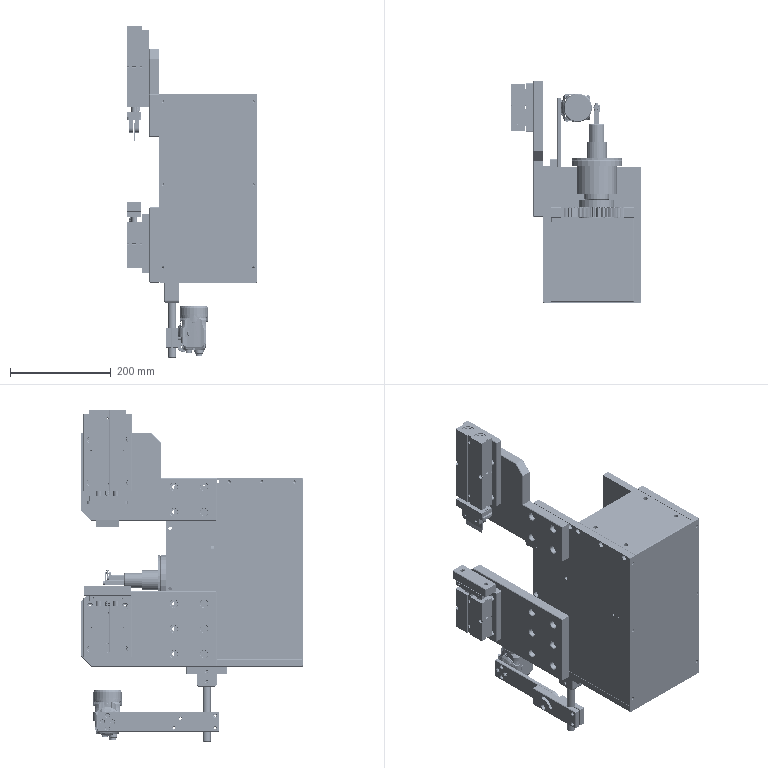Assembly | SolidWorks | mm | 54 component files | 54 solids | 5160 faces | box 260.2 x 442 x 660.5 mm | volume 8940176 mm3 | cylinder 1970 | plane 1868 | cone 912 | spline 408 | torus 2 | commonest cylinder face diameters 42 x148 8 x102 4 x85 0.4 x82 5 x74 11 x74 97.498 x70 111 x70
Bill of materials:
3M 35T | 1 | 1060 Alloy | Straight-tooth spur-gear-like disc with a cylindrical hub on one face and a keyed central bore.
BasePlate2 | 1 | 1060 Alloy | Thin rectangular, near-square plate with four through holes near the corners of the face and three holes in one edge face.
3M 35TS35B70H35L40 | 1 |  | Straight-tooth gear with a hub on one side, a large keyed bore and a ring of small holes in the web.
40ShaftRetainingRing | 1 |  | Thin flat split ring with two lugs at the gap, each with a small hole. The shape resembles an external retaining ring.
6008 GB 276-94 | 2 |  | Annular rolling-element-bearing-like assembly: an outer ring and an inner ring with a single row of balls between them.
68HoleRetainingRing | 2 |  | Thin flat open ring with two rounded lugs at the gap, each with a small hole. The shape resembles an internal retaining ring.
AirGripperFixingPlate1 | 1 | Plain Carbon Steel | Flat plate made of a circular disc joined to a rectangular tab, with a central rectangular cutout and several round holes.
AirGripperFixingPlate2 | 1 | 1060 Alloy | Rectangular block or thick plate with two round through holes.
BearingCoverPlate | 1 | Plain Carbon Steel | Thin flat annular disc with a large central hole and four small holes near the outer edge.
BearingHolder | 1 | Plain Carbon Steel | Flanged cylindrical sleeve: a hollow tube with a wider flange at one end that has a ring of holes.
Buckle | 1 |  | Push-in clip-like molded part: a wide winged head, a stem, a round disc flange, and a lower body with angled flexible-looking arms and a tip.
BuckleRotaryAxis | 1 | Plain Carbon Steel | Stepped cylindrical shaft with a raised collar, shallow ring grooves, and a rectangular socket in one end face surrounded by four small holes.
CylinderJaw1 | 1 | Plain Carbon Steel | Long straight square-section bar with an enlarged rectangular end block at one end, carrying four holes in a 2x2 pattern.
CylinderJaw2 | 1 | Plain Carbon Steel | Long straight rectangular-section bar with a rectangular end block at one end, carrying four holes in a 2x2 pattern; the block extends further below the bar than in the similar part.
FixedSleeve | 1 | Plain Carbon Steel | Short thin-walled cylindrical ring or sleeve with an open through-bore and small chamfers on the outer edges.
JawBuckleJaw | 1 | Plain Carbon Steel | Upright flat plate with a rounded top, an elongated slot near the top, a large round hole in the middle and a smaller round hole lower down; two parallel side flanges at the lower end give that section a U-channel shape.
JawBuckleJaw2 | 1 | Plain Carbon Steel | Shorter version of the flanged plate: rounded-top plate with an elongated slot above and one round hole below, and two parallel side flanges on the wider lower section forming a U-channel.
M4X16 | 3 |  | Fastener-like part: cylindrical head with a hexagonal socket recess, a short externally grooved (thread-like) section next to the head, then a longer smooth cylindrical shank of smaller diameter.
1_1_9 | 1 |  | Rectangular prismatic block with long grooves along its length, a central raised and stepped section, and several holes; the end face has two counterbored circular features.
2_13 | 1 |  | Square block plate with a large central through-hole and four corner holes, joined by a stepped offset web to a thin arm that extends sideways and ends in a small hooked lip.
3_10 | 1 |  | Square block plate with a large central hole and four corner holes, with a stepped side web and a thin arm extending the other way, ending in a small hooked lip.
SensorPlate3 | 1 | Plain Carbon Steel | L-shaped bent thin-sheet bracket with rounded outer corners and an elongated obround slot in one leg.
CameraFixingPlate | 1 | 1060 Alloy | Flat elongated plate with one fully rounded end and one square end, two holes near the rounded end and four holes in a diamond pattern near the square end.
GuideAxis16 | 1 | Plain Carbon Steel | Plain solid cylindrical rod or pin with small chamfers at both ends.
GuideAxisFixingPlate | 1 | 1060 Alloy | Stepped rectangular block with a split-clamp bore at one end and an arc slot through the thinner stepped section
GuideAxisHolder | 1 | 1060 Alloy | T-section block with a flange that has a large central bore and two flanking holes, and a downward web with two cross holes
IV-150_500_2000 | 1 |  | Complex housing with a rounded square body, a stepped circular top boss and cylindrical outlets at the bottom
OP-87436_87437 | 1 |  | Circular cap with a chamfered top, a circumferential groove and short legs or lobes below, one of which has a hole
OP-87460 | 1 |  | Curved, saddle-like bracket with a hole pattern on a central tab and a small angled flange with a hole
OP-87461 | 1 |  | Circular cap with a chamfered top, a circumferential groove, and downward legs, including a central lobe with a hole
CoverPlate4 | 1 | Plain Carbon Steel | Thin flat rectangular plate with six small holes along its two long edges
CutterBlade | 1 | Plain Carbon Steel | Flat rectangular blade-like plate with a bevel along one edge and two mounting holes
CutterFixingBlock | 1 | 1060 Alloy | Mounting bracket with a rounded-rectangle base plate and two parallel lugs with aligned cross holes
CutterFixingPlateA | 1 | 1060 Alloy | Flat rectangular plate with two chamfered corners, six larger holes and four smaller holes
CutterFixingPlateB | 1 | 1060 Alloy | L-outline flat plate with chamfered corners, four larger holes on the narrow leg and four smaller holes on the wide section
CutterNylonPad | 1 | 1060 Alloy | Rectangular block with chamfered edges and two counterbored or countersunk through-holes
Gasket5 | 1 | 1060 Alloy | Thick rectangular plate with a symmetric pattern of through holes: four larger holes and four smaller holes.
MHMJ082G1U_203 | 1 |  | Boxy body with a square flange that has four corner holes, a cylindrical shaft sticking out of one end, side-mounted connector-like housings with short bent cable stubs, and small screw heads on the end faces. Its overall form resembles a rotary motor.
SensorFixingBlock | 1 | Plain Carbon Steel | Thin L-shaped bent bracket. One leg has two round holes and the other leg has one large elongated (obround) slot.
ServoMotorFixingPlate | 1 | 1060 Alloy | Rectangular plate with a large central circular opening, four small holes around it, and four elongated slots near the short ends.
ServoMotorSideFixingPlate | 2 | 1060 Alloy | Square-section rectangular bar with two through holes on each of two adjacent faces, set at different heights.
ShimPlate4 | 1 | 1060 Alloy | Thick rectangular plate with four larger corner holes and four columns of five small holes each.
SideFixingPlate2 | 1 | 1060 Alloy | Thin flat plate with a stepped top edge (one corner area raised), two larger round holes, small holes next to them, and small holes along the top edge and side edge.
SideFixingPlate3 | 1 | 1060 Alloy | Tall rectangular block with two counterbored bores on the top end face, lengthwise grooves down the faces, T-shaped side slots, several through holes, and a small hex-shaped fitting sticking out of the bottom.
1_1_13 | 1 |  | Two parallel cylindrical rods standing on a rectangular base plate. Each rod ends in a larger-diameter cylindrical head.
2_17 | 1 |  | Shorter rectangular block with two large counterbored bores on top, a hex fitting and a small port next to them, lengthwise grooves, T-shaped side slots, and four through holes on the large face.
1_1_11 | 1 |  | Thin flat rectangular plate with many small holes in an irregular layout, grouped mostly toward one side and the top edge.
2_15 | 1 |  | Rectangular end plate holding two parallel cylindrical rods. Each rod ends in a larger cylindrical head, and the plate has two counterbored circular features and two small end holes.
TopCoverPlate | 1 | 1060 Alloy | Flat rectangular plate of uniform thickness with ten through holes: six slightly larger holes around the edge (one at each corner and one at the middle of each long edge) and four smaller plain holes set inward in an off-center rectangular pattern.
Mates:
1. coincident | BasePlate2-1 face at (-129.666, 120.264, 197.5) dir (-1, 0, 0) | SideFixingPlate3-1 face at (-129.666, 95.264, 197.5) dir (1, 0, 0)
2. concentric | BasePlate2-1 face at (-129.666, -24.736, 190) dir (-1, 0, 0) r 2.5 | SideFixingPlate3-1 face at (-144.666, -24.736, 190) dir (-1, 0, 0) r 3.3
3. concentric | BasePlate2-1 face at (-129.666, 105.264, 190) dir (-1, 0, 0) r 2.5 | SideFixingPlate3-1 face at (-144.666, 105.264, 190) dir (-1, 0, 0) r 5.5
4. coincident | BasePlate2-1 face at (35.334, 120.264, 197.5) dir (1, 0, 0) | SideFixingPlate2-1 face at (35.334, 87.764, 197.5) dir (-1, 0, 0)
5. concentric | BasePlate2-1 face at (35.334, -24.736, 190) dir (1, 0, 0) r 2.5 | SideFixingPlate2-1 face at (50.334, -24.736, 190) dir (1, 0, 0) r 5.5
6. concentric | BasePlate2-1 face at (35.334, 105.264, 190) dir (1, 0, 0) r 2.5 | SideFixingPlate2-1 face at (50.334, 105.264, 190) dir (1, 0, 0) r 5.5
7. coincident | SideFixingPlate2-1 face at (35.334, 87.764, 197.5) dir (-1, 0, 0) | ServoMotorSideFixingPlate-1 face at (35.334, 138.264, 99) dir (1, 0, 0)
8. concentric | SideFixingPlate2-1 face at (50.334, 138.264, 59) dir (1, 0, 0) r 3.4 | ServoMotorSideFixingPlate-1 face at (15.334, 138.264, 59) dir (-1, 0, 0) r 7.5
9. parallel | SideFixingPlate2-1 face at (50.334, 138.264, 139) dir (1, 0, 0) r 3.4 | ServoMotorSideFixingPlate-1 face at (15.334, 138.264, 139) dir (-1, 0, 0) r 4.5
10. coincident | SideFixingPlate3-1 face at (-129.666, 95.264, 197.5) dir (1, 0, 0) | ServoMotorSideFixingPlate-2 face at (-129.666, 138.264, 99) dir (-1, 0, 0)
11. concentric | SideFixingPlate3-1 face at (-144.666, 138.264, 59) dir (-1, 0, 0) r 3.4 | ServoMotorSideFixingPlate-2 face at (-109.666, 138.264, 59) dir (1, 0, 0) r 7.5
12. concentric | SideFixingPlate3-1 face at (-144.666, 138.264, 139) dir (-1, 0, 0) r 3.4 | ServoMotorSideFixingPlate-2 face at (-109.666, 138.264, 139) dir (1, 0, 0) r 7.5
13. coincident | ServoMotorSideFixingPlate-2 face at (-109.666, 128.264, 149) dir (0, -1, 0) | ServoMotorFixingPlate-1 face at (-47.166, 128.264, 99) dir (0, 1, 0)
14. distance | ServoMotorFixingPlate-1 face at (-129.166, 113.264, 144) dir (-1, 0, 0) | SideFixingPlate3-1 face at (-129.666, 95.264, 197.5) dir (1, 0, 0)
15. distance | ServoMotorSideFixingPlate-1 face at (15.334, 148.264, 49) dir (0, 0, -1) | ServoMotorFixingPlate-1 face at (-129.166, 113.264, 54) dir (0, 0, -1)
16. coincident | ServoMotorFixingPlate-1 face at (-47.166, 113.264, 99) dir (0, -1, 0) | MHMJ082G1U_203-1 face at (-87.166, 113.264, 139) dir (0, 1, 0)
17. concentric | MHMJ082G1U_203-1 face at (-47.166, 148.264, 99) dir (0, -1, 0) r 9.5 | 3M 35T-1 face at (-47.166, 160.264, 99) dir (0, -1, 0) r 9.5
18. parallel | MHMJ082G1U_203-1 face at (-35.166, 126.264, 96.01) dir (0, 0, -1) | 3M 35T-1 face at (-47.166, 160.264, 96) dir (0, 0, 1)
19. coincident | MHMJ082G1U_203-1 face at (-47.166, 148.264, 99) dir (0, 1, 0) | 3M 35T-1 face at (-47.166, 148.264, 99) dir (0, 1, 0)
20. concentric | ServoMotorFixingPlate-1 face at (-15.346, 113.264, 67.18) dir (0, -1, 0) r 2.1 | MHMJ082G1U_203-1 face at (-15.346, 96.778, 67.18) dir (0, 1, 0) r 3
21. concentric | ServoMotorFixingPlate-1 face at (-78.986, 113.264, 67.18) dir (0, -1, 0) r 2.1 | MHMJ082G1U_203-1 face at (-78.986, 96.778, 67.18) dir (0, 1, 0) r 3
22. coincident | SideFixingPlate3-1 face at (-144.666, 230.264, -162.5) dir (0, 0, -1) | TopCoverPlate-1 face at (-47.166, -39.736, -162.5) dir (0, 0, 1)
23. coincident | SideFixingPlate3-1 face at (-144.666, -39.736, 197.5) dir (0, -1, 0) | CoverPlate4-1 face at (-47.166, -39.736, 10) dir (0, 1, 0)
24. concentric | SideFixingPlate2-1 face at (42.834, -39.736, 182.5) dir (0, -1, 0) r 2.5 | CoverPlate4-1 face at (42.834, -39.736, 182.5) dir (0, -1, 0) r 3.5
25. concentric | SideFixingPlate3-1 face at (-137.166, -39.736, 182.5) dir (0, -1, 0) r 2.5 | CoverPlate4-1 face at (-137.166, -39.736, 182.5) dir (0, -1, 0) r 3.5
26. concentric | SideFixingPlate2-1 face at (42.834, -24.236, -162.5) dir (0, 0, -1) r 2.5 | TopCoverPlate-1 face at (42.834, -24.236, -177.5) dir (0, 0, -1) r 5.5
27. concentric | SideFixingPlate3-1 face at (-137.166, -24.236, -162.5) dir (0, 0, -1) r 2.5 | TopCoverPlate-1 face at (-137.166, -24.236, -177.5) dir (0, 0, -1) r 5.5
28. coincident | SideFixingPlate3-1 face at (-144.666, 95.264, 197.5) dir (-1, 0, 0) | CutterFixingPlateA-1 face at (-144.666, 130.264, 197.5) dir (1, 0, 0)
29. coincident | TopCoverPlate-1 face at (-47.166, -39.736, -177.5) dir (0, 0, -1) | CutterFixingPlateA-1 face at (-164.666, 130.264, -177.5) dir (0, 0, -1)
30. distance | CutterFixingPlateA-1 face at (-164.666, 130.264, 197.5) dir (0, -1, 0) | SideFixingPlate3-1 face at (-144.666, 230.264, 197.5) dir (0, 1, 0)
31. coincident | CutterFixingPlateA-1 face at (-164.666, 130.264, 197.5) dir (-1, 0, 0) | ShimPlate4-1 face at (-164.666, 347.264, -100) dir (1, 0, 0)
32. concentric | CutterFixingPlateA-1 face at (-164.666, 382.264, -142.5) dir (-1, 0, 0) r 2.5 | ShimPlate4-1 face at (-179.666, 382.264, -142.5) dir (-1, 0, 0) r 3.3
33. concentric | CutterFixingPlateA-1 face at (-164.666, 312.264, -142.5) dir (-1, 0, 0) r 2.5 | ShimPlate4-1 face at (-179.666, 312.264, -142.5) dir (-1, 0, 0) r 3.3
34. coincident | ShimPlate4-1 face at (-179.666, 347.264, -100) dir (-1, 0, 0) | TN25X30S-1/1_1_11-1 face at (-179.666, 310.614, -56) dir (1, 0, 0)
35. concentric | ShimPlate4-1 face at (-179.666, 347.264, -131) dir (-1, 0, 0) r 1.65 | TN25X30S-1/1_1_11-1 face at (-194.766, 347.264, -131) dir (1, 0, 0) r 2.25
36. concentric | ShimPlate4-1 face at (-179.666, 347.264, -71) dir (-1, 0, 0) r 1.65 | TN25X30S-1/1_1_11-1 face at (-194.766, 347.264, -71) dir (1, 0, 0) r 2.25
37. coincident | TN25X30S-1/2_15-1 face at (-180.266, 347.264, -37) dir (0, 0, 1) | CutterNylonPad-1 face at (-180.266, 300.264, -37) dir (0, 0, -1)
38. concentric | TN25X30S-1/2_15-1 face at (-194.766, 380.264, -41.5) dir (0, 0, -1) r 1.621 | CutterNylonPad-1 face at (-194.766, 380.264, -17) dir (0, 0, 1) r 4
39. concentric | TN25X30S-1/2_15-1 face at (-194.766, 314.264, -41.5) dir (0, 0, -1) r 1.621 | CutterNylonPad-1 face at (-194.766, 314.264, -17) dir (0, 0, 1) r 4
40. coincident | SideFixingPlate3-1 face at (-144.666, 95.264, 197.5) dir (-1, 0, 0) | CutterFixingPlateB-1 face at (-144.666, 130.264, 197.5) dir (1, 0, 0)
41. coincident | CutterFixingPlateA-1 face at (-164.666, 130.264, 197.5) dir (0, -1, 0) | CutterFixingPlateB-1 face at (-164.666, 130.264, 197.5) dir (0, -1, 0)
42. coincident | SideFixingPlate3-1 face at (-144.666, 230.264, 197.5) dir (0, 0, 1) | CutterFixingPlateB-1 face at (-164.666, 130.264, 197.5) dir (0, 0, 1)
43. coincident | CutterFixingPlateB-1 face at (-164.666, 130.264, 197.5) dir (-1, 0, 0) | Gasket5-1 face at (-164.666, 347.264, 248.5) dir (1, 0, 0)
44. concentric | CutterFixingPlateB-1 face at (-164.666, 312.264, 188.5) dir (-1, 0, 0) r 2.5 | Gasket5-1 face at (-179.666, 312.264, 188.5) dir (-1, 0, 0) r 3.3
45. concentric | CutterFixingPlateB-1 face at (-164.666, 382.264, 188.5) dir (-1, 0, 0) r 2.5 | Gasket5-1 face at (-179.666, 382.264, 188.5) dir (-1, 0, 0) r 3.3
46. coincident | Gasket5-1 face at (-179.666, 347.264, 248.5) dir (-1, 0, 0) | TN25X100S-1/1_1_13-1 face at (-179.666, 383.914, 171) dir (1, 0, 0)
47. concentric | Gasket5-1 face at (-179.666, 347.264, 186) dir (-1, 0, 0) r 1.65 | TN25X100S-1/1_1_13-1 face at (-206.266, 347.264, 186) dir (-1, 0, 0) r 3.75
48. concentric | Gasket5-1 face at (-179.666, 347.264, 316) dir (-1, 0, 0) r 1.65 | TN25X100S-1/1_1_13-1 face at (-194.766, 347.264, 316) dir (-1, 0, 0) r 2.25
49. coincident | TN25X100S-1/2_17-1 face at (-209.266, 347.264, 152) dir (0, 0, -1) | CutterFixingBlock-1 face at (-180.266, 387.264, 152) dir (0, 0, 1)
50. concentric | TN25X100S-1/2_17-1 face at (-194.766, 380.264, 156.5) dir (0, 0, 1) r 1.621 | CutterFixingBlock-1 face at (-194.766, 380.264, 146) dir (0, 0, -1) r 2.5
51. concentric | TN25X100S-1/2_17-1 face at (-194.766, 314.264, 156.5) dir (0, 0, 1) r 1.621 | CutterFixingBlock-1 face at (-194.766, 314.264, 146) dir (0, 0, -1) r 2.5
52. coincident | CutterFixingBlock-1 face at (-193.016, 372.264, 196.122) dir (-1, 0, 0) | CutterBlade-1 face at (-193.016, 347.264, 141) dir (1, 0, 0)
53. concentric | CutterFixingBlock-1 face at (-200.794, 362.264, 131) dir (1, 0, 0) r 2.75 | CutterBlade-1 face at (-193.016, 362.264, 131) dir (-1, 0, 0) r 2.75
54. concentric | CutterFixingBlock-1 face at (-200.794, 332.264, 131) dir (1, 0, 0) r 2.75 | CutterBlade-1 face at (-193.016, 332.264, 131) dir (-1, 0, 0) r 2.75
55. coincident | SideFixingPlate3-1 face at (-129.666, 95.264, 197.5) dir (1, 0, 0) | SensorFixingBlock-1 face at (-129.666, 17.264, 49.5) dir (-1, 0, 0)
56. concentric | SideFixingPlate3-1 face at (-129.666, 5.264, 37) dir (1, 0, 0) r 2.1 | SensorFixingBlock-1 face at (-79.666, 5.264, 37) dir (-1, 0, 0) r 2.75
57. coincident | TopCoverPlate-1 face at (-47.166, -39.736, -177.5) dir (0, 0, -1) | CameraAssembly-1/GuideAxisHolder-1 face at (-119.666, 150.264, -177.5) dir (0, 0, 1)
58. concentric | TopCoverPlate-1 face at (-119.666, 120.264, -177.5) dir (0, 0, -1) r 3.4 | CameraAssembly-1/GuideAxisHolder-1 face at (-119.666, 120.264, -192.5) dir (0, 0, -1) r 4.5
59. concentric | TopCoverPlate-1 face at (-119.666, 180.264, -177.5) dir (0, 0, -1) r 3.4 | CameraAssembly-1/GuideAxisHolder-1 face at (-119.666, 180.264, -192.5) dir (0, 0, -1) r 4.5
60. coincident | BearingHolder-1 face at (-103.056, 10.785, 121) dir (0, 0, 1) | 6008 GB 276-94-1 face at (-103.056, 44.785, 121) dir (0, 0, -1)
61. concentric | BearingHolder-1 face at (-103.056, 10.785, 121) dir (0, 0, 1) r 34 | 6008 GB 276-94-1 face at (-103.056, 10.785, 137.211) dir (0, 0, 1) r 34
62. coincident | BearingHolder-1 face at (-103.056, 10.785, 94) dir (0, 0, -1) | 6008 GB 276-94-2 face at (-103.056, 44.785, 94) dir (0, 0, 1)
63. concentric | BearingHolder-1 face at (-103.056, 10.785, 94) dir (0, 0, -1) r 34 | 6008 GB 276-94-2 face at (-103.056, 10.785, 77.789) dir (0, 0, -1) r 34
64. concentric | BearingHolder-1 face at (-103.056, 10.785, 141) dir (0, 0, -1) r 40 | 68HoleRetainingRing-1 face at (-103.056, 10.785, 136) dir (0, 0, 1) r 36.25
65. coincident | BearingHolder-1 face at (-103.056, 44.785, 136) dir (0, 0, 1) | 68HoleRetainingRing-1 face at (-103.056, 10.785, 136) dir (0, 0, -1)
66. concentric | BearingHolder-1 face at (-103.056, 10.785, 86) dir (0, 0, -1) r 50 | 68HoleRetainingRing-2 face at (-103.056, 10.785, 76.5) dir (0, 0, 1) r 36.25
67. coincident | BearingHolder-1 face at (-103.056, 44.785, 79) dir (0, 0, -1) | 68HoleRetainingRing-2 face at (-103.056, 10.785, 79) dir (0, 0, 1)
68. concentric | 6008 GB 276-94-2 face at (-103.056, 10.785, 79.529) dir (0, 0, -1) r 20 | BuckleRotaryAxis-1 face at (-103.056, 10.785, 37) dir (0, 0, 1) r 20
69. coincident | 6008 GB 276-94-2 face at (-103.056, 35.452, 79) dir (0, 0, -1) | BuckleRotaryAxis-1 face at (-123.056, 10.785, 79) dir (0, 0, -1)
70. coincident | BuckleRotaryAxis-1 face at (-123.056, 10.785, 79) dir (0, 0, -1) | 40ShaftRetainingRing-1 face at (-102.577, 9.63, 79) dir (0, 0, 1)
71. concentric | BuckleRotaryAxis-1 face at (-103.056, 10.785, 37) dir (0, 0, 1) r 20 | 40ShaftRetainingRing-1 face at (-103.056, 10.785, 79) dir (0, 0, -1) r 22
72. angle | BearingHolder-1 plane at (-103.056, 10.785, 74) dir (1, 0, 0) | BuckleRotaryAxis-1 face at (-108.056, 20.785, 187) dir (1, 0, 0)
73. concentric | BuckleRotaryAxis-1 face at (-103.056, 10.785, 37) dir (0, 0, 1) r 20 | FixedSleeve-1 face at (-103.056, 10.785, 121) dir (0, 0, -1) r 25
74. coincident | 6008 GB 276-94-1 face at (-103.056, 30.785, 121) dir (0, 0, -1) | FixedSleeve-1 face at (-103.056, 10.785, 121) dir (0, 0, 1)
75. concentric | BuckleRotaryAxis-1 face at (-103.056, 10.785, 152) dir (0, 0, 1) r 20 | 3M 35TS35B70H35L40-1 face at (-103.056, 10.785, 202) dir (0, 0, -1) r 20
76. coincident | BuckleRotaryAxis-1 face at (-103.056, 10.785, 187) dir (0, 0, 1) | 3M 35TS35B70H35L40-1 face at (-103.056, 10.785, 187) dir (0, 0, 1)
77. coincident | 3M 35TS35B70H35L40-1 face at (-103.056, 10.785, 187) dir (0, 0, 1) | AirGripperFixingPlate1-1 face at (-103.056, 10.785, 187) dir (0, 0, -1)
78. coincident | AirGripperFixingPlate1-1 face at (-103.056, 10.785, 195) dir (0, 0, 1) | AirGripperFixingPlate2-1 face at (-141.056, -29.215, 195) dir (0, 0, -1)
79. concentric | AirGripperFixingPlate1-1 face at (-146.056, -6.715, 187) dir (0, 0, -1) r 3.3 | AirGripperFixingPlate2-1 face at (-146.056, -6.715, 195) dir (0, 0, -1) r 2.1
80. concentric | AirGripperFixingPlate1-1 face at (-146.056, 28.285, 187) dir (0, 0, -1) r 3.3 | AirGripperFixingPlate2-1 face at (-146.056, 28.285, 195) dir (0, 0, -1) r 2.1
81. concentric | 3M 35TS35B70H35L40-1 face at (-68.056, 10.785, 187) dir (0, 0, 1) r 2.1 | AirGripperFixingPlate1-1 face at (-68.056, 10.785, 195) dir (0, 0, 1) r 5
82. coincident | AirGripperFixingPlate2-1 face at (-141.056, 10.785, 195) dir (1, 0, 0) | MHF2-16D_16_0-1/1_1_9-1 face at (-141.056, -10.215, 275) dir (-1, 0, 0)
83. concentric | AirGripperFixingPlate2-1 face at (-151.056, -2.715, 220) dir (-1, 0, 0) r 2.75 | MHF2-16D_16_0-1/1_1_9-1 face at (-134.539, -2.715, 220) dir (1, 0, 0) r 2.067
84. concentric | AirGripperFixingPlate2-1 face at (-151.056, -2.715, 258) dir (-1, 0, 0) r 2.75 | MHF2-16D_16_0-1/1_1_9-1 face at (-134.539, -2.715, 258) dir (1, 0, 0) r 2.067
85. coincident | MHF2-16D_16_0-1/2_13-1 face at (-108.056, -16.215, 236) dir (1, 0, 0) | CylinderJaw1-1 face at (-108.056, 10.785, 234.8) dir (-1, 0, 0)
86. concentric | MHF2-16D_16_0-1/2_13-1 face at (-110.245, 7.285, 229.8) dir (1, 0, 0) r 1.621 | CylinderJaw1-1 face at (-98.056, 7.285, 229.8) dir (1, 0, 0) r 2.25
87. concentric | MHF2-16D_16_0-1/2_13-1 face at (-110.245, -12.715, 229.8) dir (1, 0, 0) r 1.621 | CylinderJaw1-1 face at (-98.056, -12.715, 229.8) dir (1, 0, 0) r 2.25
88. coincident | MHF2-16D_16_0-1/3_10-1 face at (-108.056, 10.785, 242) dir (1, 0, 0) | CylinderJaw2-1 face at (-108.056, 20.785, 268.2) dir (-1, 0, 0)
89. concentric | MHF2-16D_16_0-1/3_10-1 face at (-110.245, 7.285, 263.2) dir (1, 0, 0) r 1.621 | CylinderJaw2-1 face at (-98.056, 7.285, 263.2) dir (1, 0, 0) r 2.25
90. concentric | MHF2-16D_16_0-1/3_10-1 face at (-110.245, -12.715, 263.2) dir (1, 0, 0) r 1.621 | CylinderJaw2-1 face at (-98.056, -12.715, 263.2) dir (1, 0, 0) r 2.25
91. coincident | AirGripperFixingPlate1-1 face at (-91.035, -3.486, 190.4) dir (0, 0, 1) | M4X16-1 face at (-91.035, -1.236, 190.4) dir (0, 0, -1)
92. concentric | AirGripperFixingPlate1-1 face at (-91.035, -1.236, 195) dir (0, 0, 1) r 4 | M4X16-1 face at (-91.035, -1.236, 190.4) dir (0, 0, 1) r 3.5
93. coincident | CylinderJaw1-1 face at (-98.056, 10.785, -33.2) dir (0, 0, -1) | JawBuckleJaw-1 face at (-103.056, 0.7849, -33.2) dir (0, 0, 1)
94. concentric | CylinderJaw1-1 face at (-103.056, 5.785, -33.2) dir (0, 0, -1) r 1.65 | JawBuckleJaw-1 face at (-103.056, 5.785, -33.2) dir (0, 0, 1) r 2.25
95. coincident | CylinderJaw1-1 face at (-98.056, 10.785, 234.8) dir (1, 0, 0) | JawBuckleJaw-1 face at (-98.056, 10.785, -36.2) dir (-1, 0, 0)
96. concentric | BearingHolder-1 face at (-103.056, 10.785, 141) dir (0, 0, -1) r 40 | AirGripperFixingPlate1-1 face at (-103.056, 10.785, 195) dir (0, 0, -1) r 42.5
97. coincident | CylinderJaw2-1 face at (-98.056, 20.785, -24.8) dir (0, 0, -1) | JawBuckleJaw2-1 face at (-103.056, 10.785, -24.8) dir (0, 0, 1)
98. concentric | CylinderJaw2-1 face at (-103.056, 15.785, -24.8) dir (0, 0, -1) r 1.65 | JawBuckleJaw2-1 face at (-103.056, 15.785, -24.8) dir (0, 0, 1) r 2.25
99. coincident | CylinderJaw2-1 face at (-98.056, 20.785, 268.2) dir (1, 0, 0) | JawBuckleJaw2-1 face at (-98.056, 20.785, -27.8) dir (-1, 0, 0)
100. concentric | JawBuckleJaw2-1 face at (-103.056, 15.785, -24.8) dir (0, 0, 1) r 2.25 | M4X16-2 face at (-103.056, 15.785, -27.8) dir (0, 0, -1) r 3.5
101. coincident | JawBuckleJaw2-1 face at (-103.056, 10.785, -27.8) dir (0, 0, -1) | M4X16-2 face at (-103.056, 15.785, -27.8) dir (0, 0, 1)
102. concentric | JawBuckleJaw-1 face at (-103.056, 5.785, -33.2) dir (0, 0, 1) r 2.25 | M4X16-3 face at (-103.056, 5.785, -36.2) dir (0, 0, -1) r 3.5
103. coincident | JawBuckleJaw-1 face at (-103.056, 0.7849, -36.2) dir (0, 0, -1) | M4X16-3 face at (-103.056, 5.785, -36.2) dir (0, 0, 1)
104. coincident | BearingHolder-1 face at (-103.056, 10.785, 74) dir (0, 0, -1) | BearingCoverPlate-1 face at (-103.056, 10.785, 74) dir (0, 0, 1)
105. concentric | BearingHolder-1 face at (-63.178, 29.38, 74) dir (0, 0, -1) r 2.1 | BearingCoverPlate-1 face at (-63.178, 29.38, 69) dir (0, 0, 1) r 3
106. concentric | BearingHolder-1 face at (-121.651, 50.662, 74) dir (0, 0, -1) r 2.1 | BearingCoverPlate-1 face at (-121.651, 50.662, 69) dir (0, 0, 1) r 3
107. coincident | JawBuckleJaw2-1 face at (-98.056, 27.785, -27.8) dir (0, 1, 0) | Buckle-1 face at (-105.281, 27.785, -28.025) dir (0, -1, 0)
108. distance | Buckle-1 plane at (-103.056, 25.81, -30.7) dir (0, 0, -1) | JawBuckleJaw-1 face at (-103.056, 0.7849, -33.2) dir (0, 0, 1)
109. coincident | JawBuckleJaw-1 plane at (-103.056, 0.7849, -33.2) dir (1, 0, 0) | Buckle-1 plane at (-103.056, 25.81, -30.7) dir (-1, 0, 0)
110. coincident | AirGripperFixingPlate2-1 face at (-141.056, -29.215, 195) dir (0, -1, 0) | SensorPlate3-1 face at (-141.056, -29.215, 255) dir (0, 1, 0)
111. coincident | AirGripperFixingPlate2-1 face at (-141.056, 10.785, 195) dir (1, 0, 0) | SensorPlate3-1 face at (-141.056, -29.215, 275) dir (1, 0, 0)
112. coincident | AirGripperFixingPlate2-1 face at (-141.056, -29.215, 275) dir (0, 0, 1) | SensorPlate3-1 face at (-141.056, -29.215, 275) dir (0, 0, 1)
113. distance | 3_10-1 face at (0, -33, 30.4) dir (0, 0, 1) | 1_1_9-1 face at (0, 0, 36) dir (0, 0, 1)
114. coincident | 1_1_9-1 face at (-6.1, -28.3, 36) dir (0, -1, 0) | 3_10-1 face at (-6.1, -28.3, 8) dir (0, 1, 0)
115. coincident | 1_1_9-1 face at (6.1, -28.3, 36) dir (1, 0, 0) | 3_10-1 face at (6.1, -28.3, 8) dir (-1, 0, 0)
116. distance | 1_1_9-1 face at (0, 0, -36) dir (0, 0, -1) | 2_13-1 face at (0, -33, -30.4) dir (0, 0, -1)
117. coincident | 1_1_9-1 face at (-6.1, -28.3, 36) dir (0, -1, 0) | 2_13-1 face at (6.1, -28.3, -8) dir (0, 1, 0)
118. coincident | 1_1_9-1 face at (-6.1, -20, 36) dir (-1, 0, 0) | 2_13-1 face at (-6.1, -28.3, -8) dir (1, 0, 0)
119. concentric | GuideAxisHolder-1 face at (5.247, -15.124, 60) dir (0, 0, 1) r 8 | GuideAxis16-1 face at (5.247, -15.124, 210) dir (0, 0, -1) r 8
120. coincident | GuideAxisHolder-1 face at (5.247, -15.124, 60) dir (0, 0, -1) | GuideAxis16-1 face at (5.247, -15.124, 60) dir (0, 0, -1)
121. concentric | GuideAxis16-1 face at (5.247, -15.124, 210) dir (0, 0, -1) r 8 | GuideAxisFixingPlate-1 face at (5.247, -15.124, 150) dir (0, 0, 1) r 8
122. distance | GuideAxis16-1 face at (5.247, -15.124, 210) dir (0, 0, 1) | GuideAxisFixingPlate-1 face at (-19.753, -15.124, 190) dir (0, 0, 1)
123. parallel | GuideAxisHolder-1 face at (-34.753, -30.124, 100) dir (0, -1, 0) | GuideAxisFixingPlate-1 face at (-19.753, -27.624, 190) dir (0, -1, 0)
124. coincident | GuideAxisFixingPlate-1 face at (100.247, -12.624, 150) dir (0, 1, 0) | CameraFixingPlate-1 face at (45.247, -12.624, 170) dir (0, -1, 0)
125. concentric | GuideAxisFixingPlate-1 face at (70.247, -27.624, 182) dir (0, -1, 0) r 3.3 | CameraFixingPlate-1 face at (70.247, -12.624, 182) dir (0, -1, 0) r 2.5
126. angle | GuideAxisFixingPlate-1 face at (-19.753, -15.124, 190) dir (0, 0, 1) | CameraFixingPlate-1 face at (45.247, -12.624, 190) dir (0, 0, 1)
127. coincident | CameraFixingPlate-1 face at (45.247, -4.624, 170) dir (0, 1, 0) | IV-150_500_OP-87436_2-1/OP-87460-1 face at (202.247, -4.624, 182.5) dir (0, -1, 0)
128. concentric | CameraFixingPlate-1 face at (202.247, -12.624, 182.5) dir (0, -1, 0) r 4 | IV-150_500_OP-87436_2-1/OP-87460-1 face at (202.247, 1.376, 182.5) dir (0, -1, 0) r 2
129. concentric | CameraFixingPlate-1 face at (202.247, -12.624, 157.5) dir (0, -1, 0) r 4 | IV-150_500_OP-87436_2-1/OP-87460-1 face at (202.247, 1.376, 157.5) dir (0, -1, 0) r 2
130. distance | 2_17-1 face at (-19, 0, -0.6) dir (-1, 0, 0) | 1_1_13-1 face at (0, 0, 0) dir (-1, 0, 0)
131. concentric | 1_1_13-1 face at (0.9, -17, -15.1) dir (1, 0, 0) r 12.5 | 2_17-1 face at (-24.6, -17, -15.1) dir (1, 0, 0) r 6
132. concentric | 1_1_13-1 face at (0.9, 17, -15.1) dir (1, 0, 0) r 12.5 | 2_17-1 face at (-24.6, 17, -15.1) dir (1, 0, 0) r 6
133. distance | 2_15-1 face at (-19, 0, -0.6) dir (-1, 0, 0) | 1_1_11-1 face at (0, 0, 0) dir (-1, 0, 0)
134. concentric | 1_1_11-1 face at (0.9, -17, -15.1) dir (1, 0, 0) r 12.5 | 2_15-1 face at (30.4, -17, -15.1) dir (1, 0, 0) r 6
135. concentric | 1_1_11-1 face at (0.9, 17, -15.1) dir (1, 0, 0) r 12.5 | 2_15-1 face at (30.4, 17, -15.1) dir (1, 0, 0) r 6